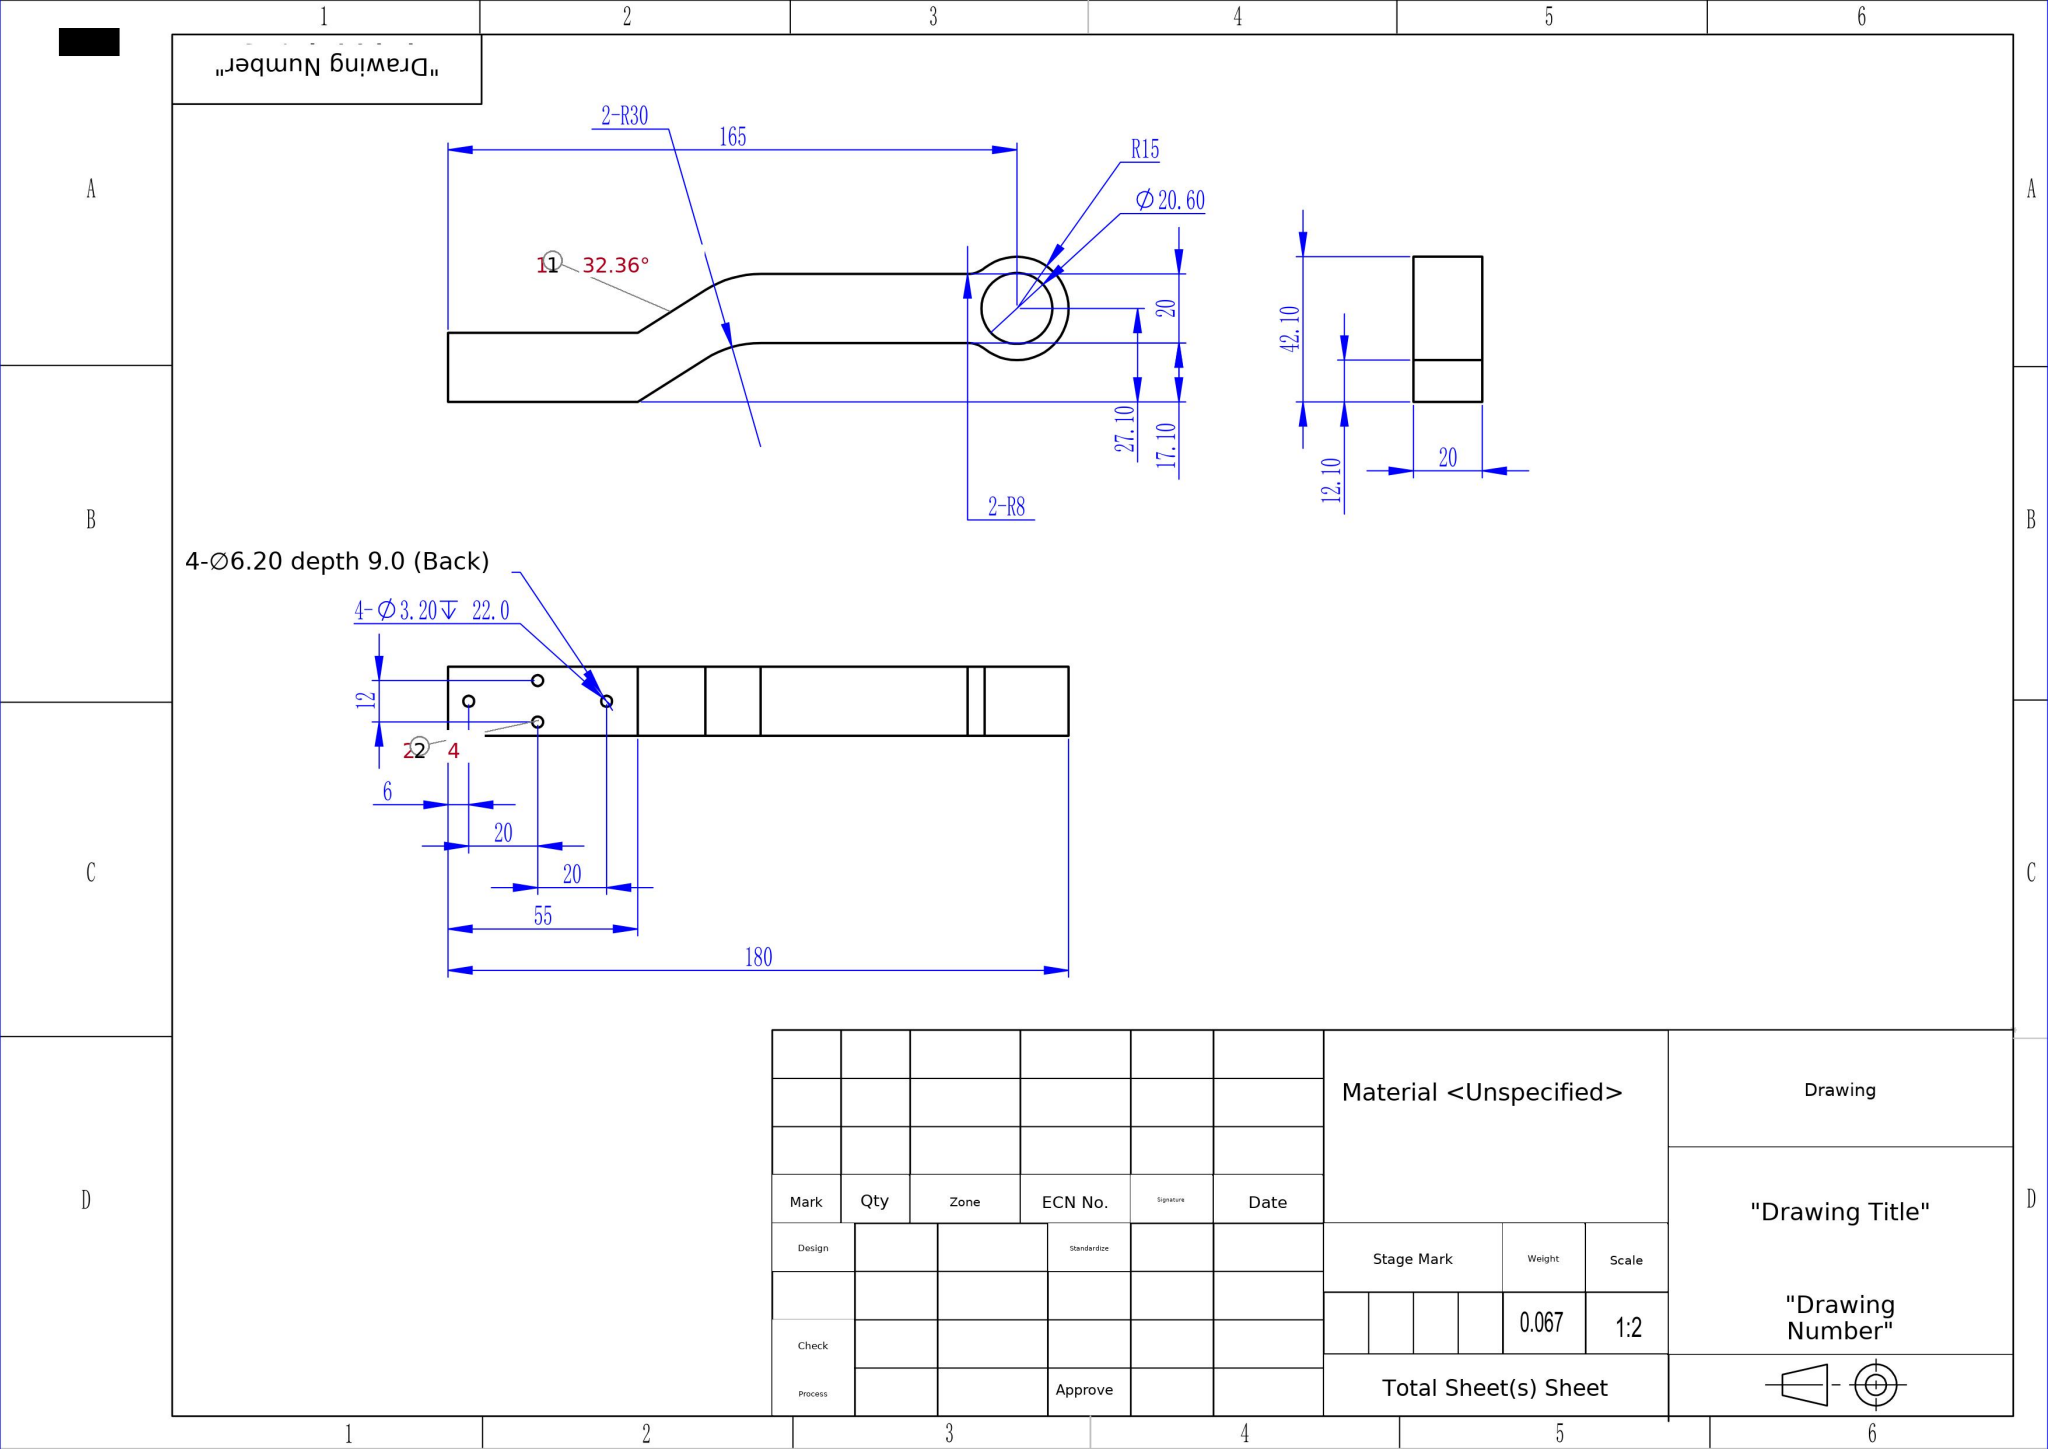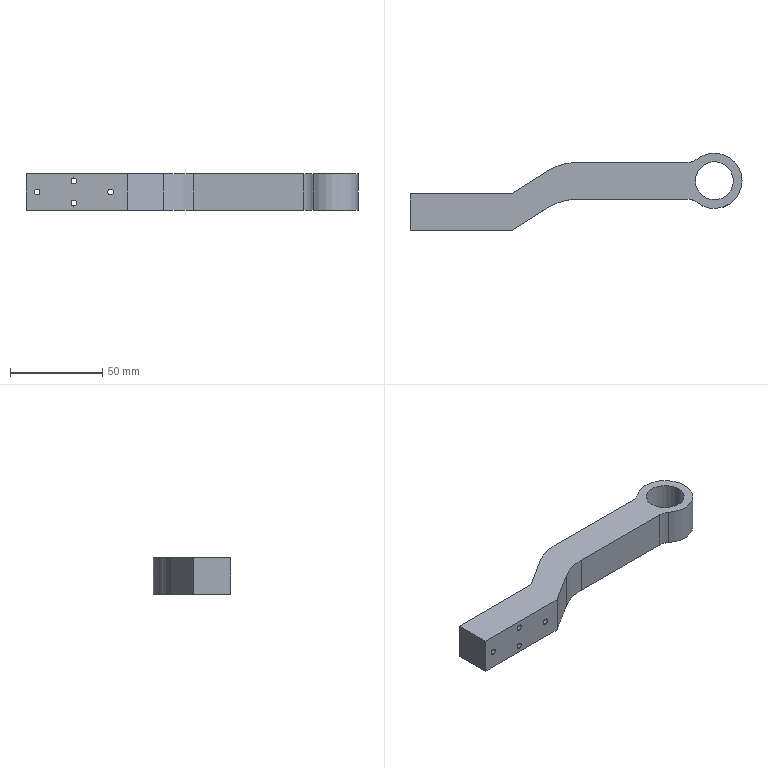Part | SolidWorks | mm | 1 solid | 36 faces | box 180 x 42.1 x 20 mm | volume 66552 mm3 | cylinder 23 | plane 13 | commonest cylinder face diameters 6.2 x8 3.2 x8 20.6 x2 16 x2 60 x2 30 x1
build123d program:
from build123d import *

# Parameters (mm, degrees)
MODEL_R             = 10.3
BOSS_EXTRUDE1_DEPTH = 20
SKETCH2_R           = 1.6
CUT_EXTRUDE1_DEPTH  = 22
SKETCH4_R           = 3.1
CUT_EXTRUDE2_DEPTH  = 9
SKETCH5_W           = 3
SKETCH5_H           = 20
CUT_EXTRUDE3_DEPTH  = 22


with BuildPart() as part:
    # Model → Boss-Extrude1 (new body)
    with BuildSketch(Plane.XY):
        with BuildLine():
            Line((233.591, 295.284), (226.238, 290.624))
            Line((226.238, 290.624), (217.532, 290.624))
            Line((217.532, 290.624), (168.238, 290.624))
            Line((168.238, 290.624), (168.238, 270.624))
            Line((168.238, 270.624), (226.238, 270.624))
            Line((226.238, 270.624), (245.869, 283.065))
            ThreePointArc((245.869, 283.065), (253.567, 286.536), (261.928, 287.725))
            Line((261.928, 287.725), (321.919, 287.725))
            ThreePointArc((321.919, 287.725), (324.556, 287.278), (326.899, 285.985))
            ThreePointArc((326.899, 285.985), (351.238, 297.723), (326.9, 309.463))
            ThreePointArc((326.9, 309.463), (324.558, 308.171), (321.92, 307.724))
            Line((321.92, 307.724), (261.928, 307.725))
            ThreePointArc((261.928, 307.725), (253.567, 306.536), (245.869, 303.065))
            Line((245.869, 303.065), (233.591, 295.284))
        make_face()
        with Locations((336.238, 297.724)):
            Circle(MODEL_R, mode=Mode.SUBTRACT)
    extrude(amount=BOSS_EXTRUDE1_DEPTH)

    # Sketch2 → Cut-Extrude1 (cut)
    with BuildSketch(Plane(origin=(0, 270.624, 0), x_dir=(-1, 0, 0), z_dir=(0, -1, 0))):
        with Locations(Location((-177.238, -10, 0), (0, 0, 90))):
            Circle(SKETCH2_R)
        with Locations(Location((-217.238, -10, 0), (0, 0, 90))):
            Circle(SKETCH2_R)
        with Locations(Location((-197.238, -16, 0), (0, 0, 90))):
            Circle(SKETCH2_R)
        with Locations(Location((-197.238, -4, 0), (0, 0, 90))):
            Circle(SKETCH2_R)
    extrude(amount=-CUT_EXTRUDE1_DEPTH, mode=Mode.SUBTRACT)

    # Sketch4 → Cut-Extrude2 (cut)
    with BuildSketch(Plane(origin=(0, 290.624, 0), x_dir=(1, 0, 0), z_dir=(0, 1, 0))):
        with Locations(Location((177.238, -10, 0), (0, 0, 270))):
            Circle(SKETCH4_R)
        with Locations(Location((197.238, -16, 0), (0, 0, 270))):
            Circle(SKETCH4_R)
        with Locations(Location((197.238, -4, 0), (0, 0, 270))):
            Circle(SKETCH4_R)
        with Locations(Location((217.238, -10, 0), (0, 0, 270))):
            Circle(SKETCH4_R)
    extrude(amount=-CUT_EXTRUDE2_DEPTH, mode=Mode.SUBTRACT)

    # Sketch5 → Cut-Extrude3 (cut)
    with BuildSketch(Plane(origin=(0, 290.624, 0), x_dir=(1, 0, 0), z_dir=(0, 1, 0))):
        with Locations((169.738, -10)):
            Rectangle(SKETCH5_W, SKETCH5_H)
    extrude(amount=-CUT_EXTRUDE3_DEPTH, mode=Mode.SUBTRACT)


solid = part.part